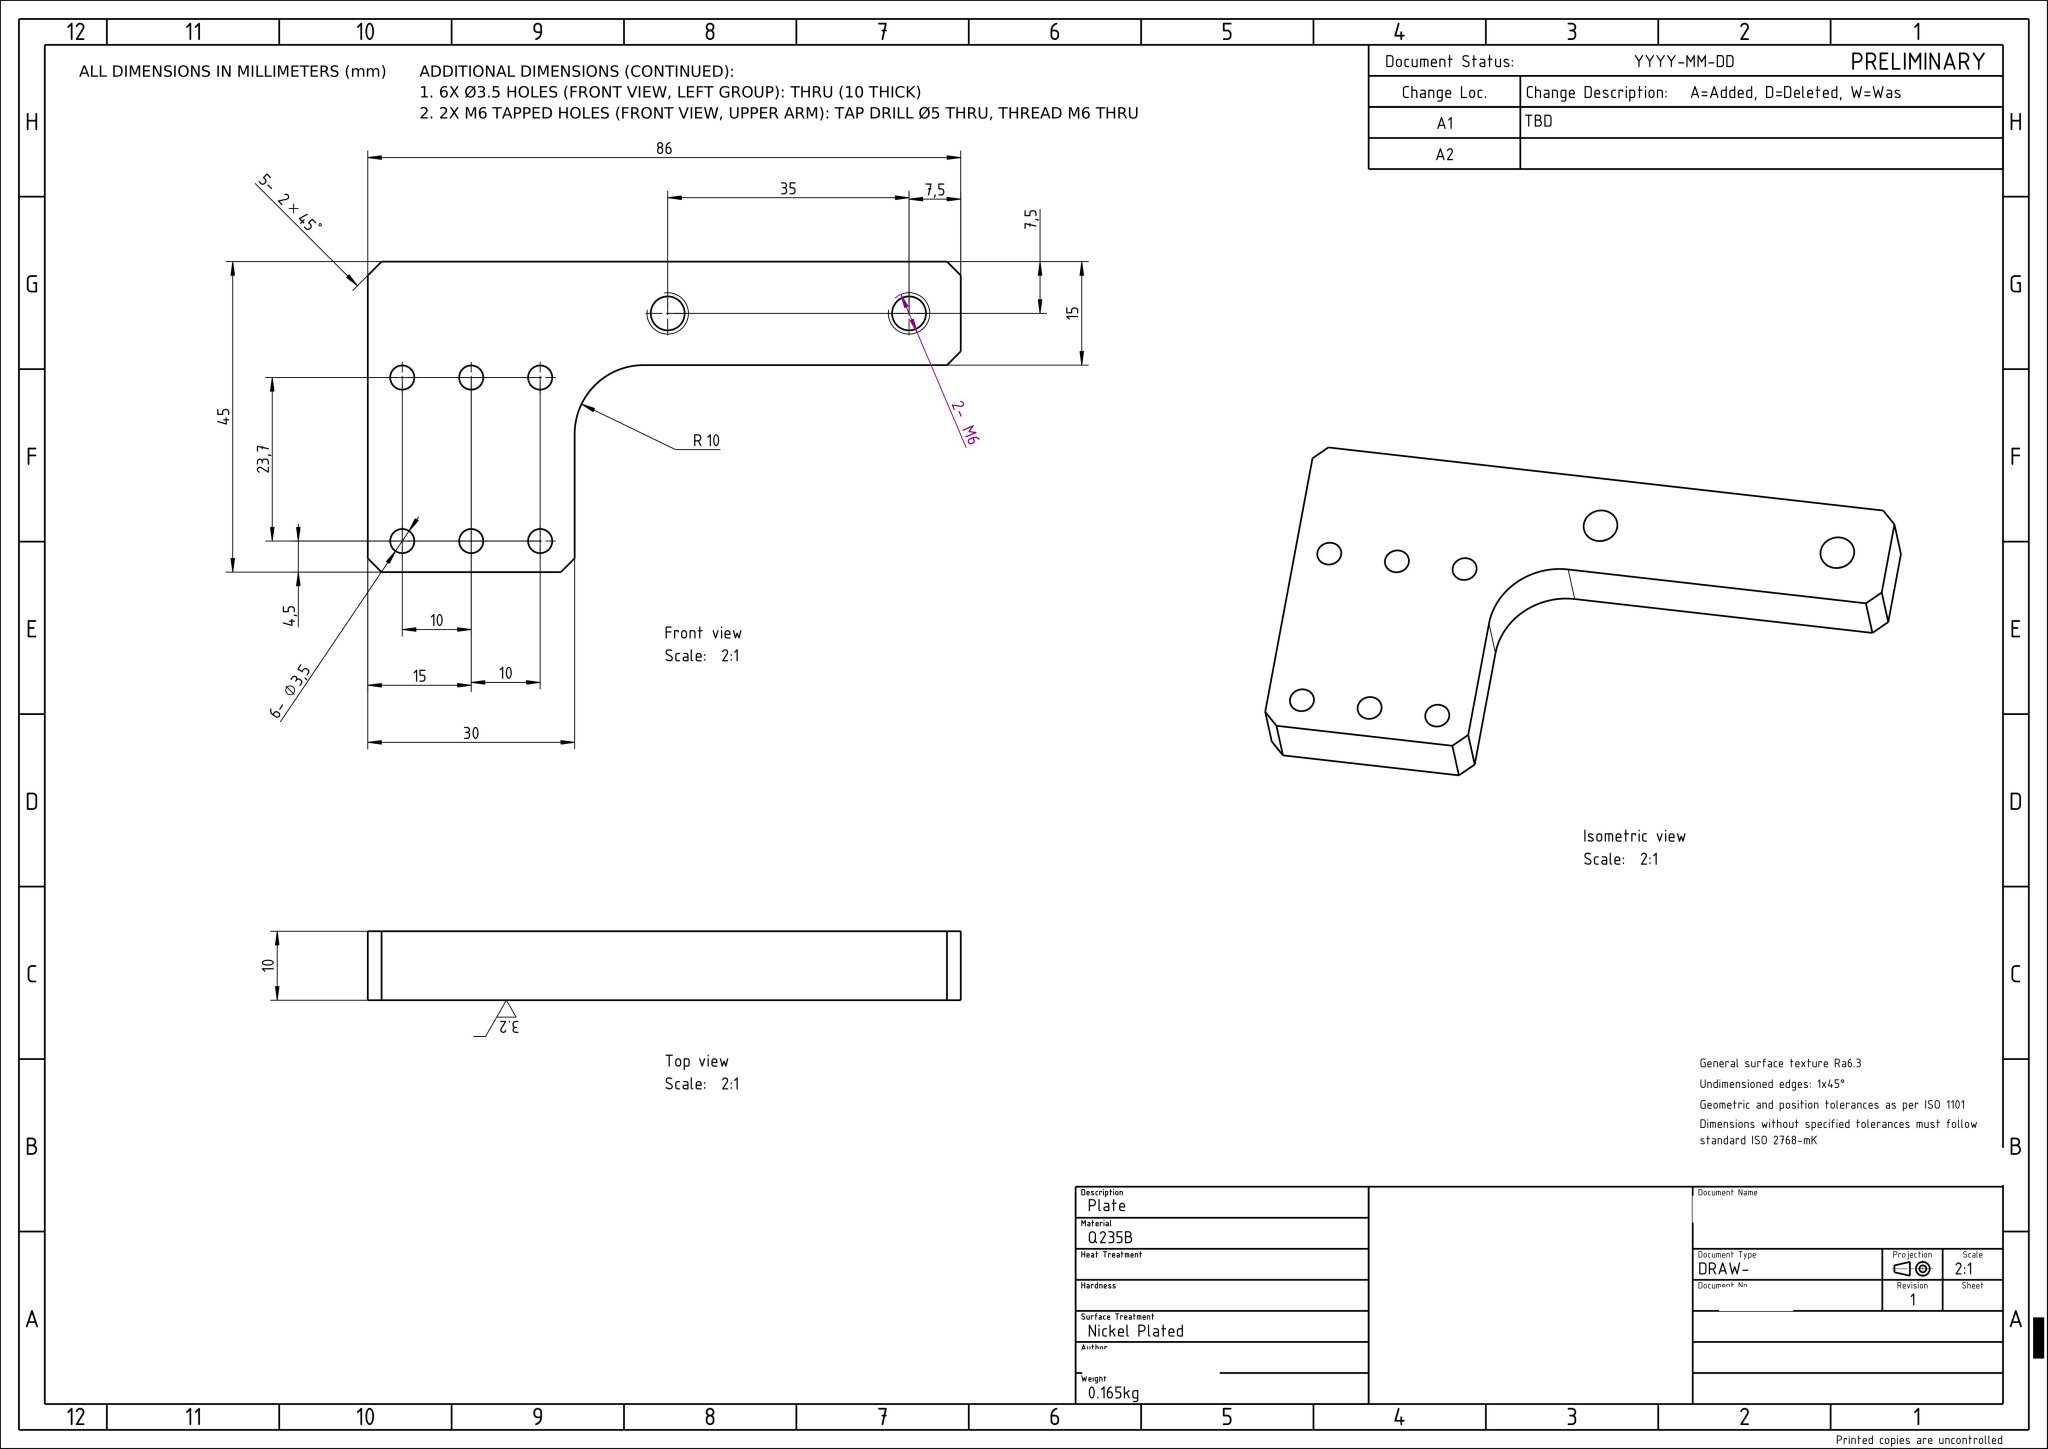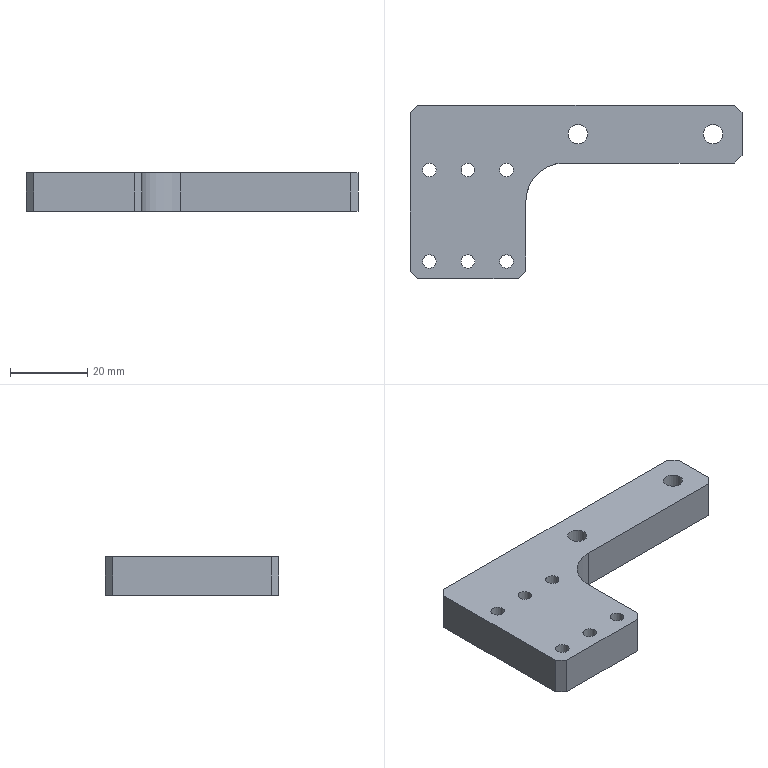Part | NX | mm | 1 solid | 22 faces | box 86 x 45 x 10 mm | volume 21045 mm3 | plane 13 | cylinder 9 | commonest cylinder face diameters 3.5 x6 5 x2 20 x1
STEP:
#1=CARTESIAN_POINT('',(0.,0.,0.));
#2=DIRECTION('',(0.,0.,1.));
#3=DIRECTION('',(1.,0.,0.));
#4=AXIS2_PLACEMENT_3D('',#1,#2,#3);
#5=(LENGTH_UNIT()NAMED_UNIT(*)SI_UNIT(.MILLI.,.METRE.));
#6=UNCERTAINTY_MEASURE_WITH_UNIT(LENGTH_MEASURE(0.00002),#5,'','');
#7=(NAMED_UNIT(*)PLANE_ANGLE_UNIT()SI_UNIT($,.RADIAN.));
#8=PLANE_ANGLE_MEASURE_WITH_UNIT(PLANE_ANGLE_MEASURE(0.01745),#7);
#9=DIMENSIONAL_EXPONENTS(0.,0.,0.,0.,0.,0.,0.);
#10=(CONVERSION_BASED_UNIT('',#8)NAMED_UNIT(#9)PLANE_ANGLE_UNIT());
#11=(NAMED_UNIT(*)SI_UNIT($,.STERADIAN.)SOLID_ANGLE_UNIT());
#12=(GEOMETRIC_REPRESENTATION_CONTEXT(3)GLOBAL_UNCERTAINTY_ASSIGNED_CONTEXT((#6))GLOBAL_UNIT_ASSIGNED_CONTEXT((#5,#10,#11))REPRESENTATION_CONTEXT('',''));
#13=SHAPE_REPRESENTATION('',(#4),#12);
#14=CARTESIAN_POINT('',(-15.,20.5,10.));
#15=VERTEX_POINT('',#14);
#16=CARTESIAN_POINT('',(-15.,-20.5,10.));
#17=VERTEX_POINT('',#16);
#18=CARTESIAN_POINT('',(-15.,22.5,10.));
#19=DIRECTION('',(-0.,-1.,0.));
#20=VECTOR('',#19,1.);
#21=LINE('',#18,#20);
#22=EDGE_CURVE('',#15,#17,#21,.T.);
#23=ORIENTED_EDGE('',*,*,#22,.F.);
#24=CARTESIAN_POINT('',(-15.,20.5,0.));
#25=VERTEX_POINT('',#24);
#26=CARTESIAN_POINT('',(-15.,20.5,10.));
#27=DIRECTION('',(0.,0.,-1.));
#28=VECTOR('',#27,1.);
#29=LINE('',#26,#28);
#30=EDGE_CURVE('',#15,#25,#29,.T.);
#31=ORIENTED_EDGE('',*,*,#30,.T.);
#32=CARTESIAN_POINT('',(-15.,-20.5,0.));
#33=VERTEX_POINT('',#32);
#34=CARTESIAN_POINT('',(-15.,22.5,0.));
#35=DIRECTION('',(-0.,-1.,0.));
#36=VECTOR('',#35,1.);
#37=LINE('',#34,#36);
#38=EDGE_CURVE('',#25,#33,#37,.T.);
#39=ORIENTED_EDGE('',*,*,#38,.T.);
#40=CARTESIAN_POINT('',(-15.,-20.5,10.));
#41=DIRECTION('',(0.,0.,1.));
#42=VECTOR('',#41,1.);
#43=LINE('',#40,#42);
#44=EDGE_CURVE('',#33,#17,#43,.T.);
#45=ORIENTED_EDGE('',*,*,#44,.T.);
#46=EDGE_LOOP('',(#23,#31,#39,#45));
#47=FACE_OUTER_BOUND('',#46,.T.);
#48=CARTESIAN_POINT('',(-15.,22.5,10.));
#49=DIRECTION('',(1.,-0.,0.));
#50=DIRECTION('',(0.,1.,0.));
#51=AXIS2_PLACEMENT_3D('',#48,#49,#50);
#52=PLANE('',#51);
#53=ADVANCED_FACE('',(#47),#52,.F.);
#54=CARTESIAN_POINT('',(-13.,-22.5,0.));
#55=VERTEX_POINT('',#54);
#56=CARTESIAN_POINT('',(13.,-22.5,0.));
#57=VERTEX_POINT('',#56);
#58=CARTESIAN_POINT('',(-15.,-22.5,0.));
#59=DIRECTION('',(1.,-0.,0.));
#60=VECTOR('',#59,1.);
#61=LINE('',#58,#60);
#62=EDGE_CURVE('',#55,#57,#61,.T.);
#63=ORIENTED_EDGE('',*,*,#62,.T.);
#64=CARTESIAN_POINT('',(13.,-22.5,10.));
#65=VERTEX_POINT('',#64);
#66=CARTESIAN_POINT('',(13.,-22.5,10.));
#67=DIRECTION('',(0.,0.,1.));
#68=VECTOR('',#67,1.);
#69=LINE('',#66,#68);
#70=EDGE_CURVE('',#57,#65,#69,.T.);
#71=ORIENTED_EDGE('',*,*,#70,.T.);
#72=CARTESIAN_POINT('',(-13.,-22.5,10.));
#73=VERTEX_POINT('',#72);
#74=CARTESIAN_POINT('',(-15.,-22.5,10.));
#75=DIRECTION('',(1.,-0.,0.));
#76=VECTOR('',#75,1.);
#77=LINE('',#74,#76);
#78=EDGE_CURVE('',#73,#65,#77,.T.);
#79=ORIENTED_EDGE('',*,*,#78,.F.);
#80=CARTESIAN_POINT('',(-13.,-22.5,10.));
#81=DIRECTION('',(0.,0.,-1.));
#82=VECTOR('',#81,1.);
#83=LINE('',#80,#82);
#84=EDGE_CURVE('',#73,#55,#83,.T.);
#85=ORIENTED_EDGE('',*,*,#84,.T.);
#86=EDGE_LOOP('',(#63,#71,#79,#85));
#87=FACE_OUTER_BOUND('',#86,.T.);
#88=CARTESIAN_POINT('',(-15.,-22.5,10.));
#89=DIRECTION('',(0.,1.,0.));
#90=DIRECTION('',(-1.,0.,0.));
#91=AXIS2_PLACEMENT_3D('',#88,#89,#90);
#92=PLANE('',#91);
#93=ADVANCED_FACE('',(#87),#92,.F.);
#94=CARTESIAN_POINT('',(15.,-20.5,10.));
#95=VERTEX_POINT('',#94);
#96=CARTESIAN_POINT('',(15.,-2.5,10.));
#97=VERTEX_POINT('',#96);
#98=CARTESIAN_POINT('',(15.,-22.5,10.));
#99=DIRECTION('',(0.,1.,0.));
#100=VECTOR('',#99,1.);
#101=LINE('',#98,#100);
#102=EDGE_CURVE('',#95,#97,#101,.T.);
#103=ORIENTED_EDGE('',*,*,#102,.F.);
#104=CARTESIAN_POINT('',(15.,-20.5,0.));
#105=VERTEX_POINT('',#104);
#106=CARTESIAN_POINT('',(15.,-20.5,10.));
#107=DIRECTION('',(0.,0.,-1.));
#108=VECTOR('',#107,1.);
#109=LINE('',#106,#108);
#110=EDGE_CURVE('',#95,#105,#109,.T.);
#111=ORIENTED_EDGE('',*,*,#110,.T.);
#112=CARTESIAN_POINT('',(15.,-2.5,0.));
#113=VERTEX_POINT('',#112);
#114=CARTESIAN_POINT('',(15.,-22.5,0.));
#115=DIRECTION('',(0.,1.,0.));
#116=VECTOR('',#115,1.);
#117=LINE('',#114,#116);
#118=EDGE_CURVE('',#105,#113,#117,.T.);
#119=ORIENTED_EDGE('',*,*,#118,.T.);
#120=CARTESIAN_POINT('',(15.,-2.5,10.));
#121=DIRECTION('',(0.,0.,1.));
#122=VECTOR('',#121,1.);
#123=LINE('',#120,#122);
#124=EDGE_CURVE('',#113,#97,#123,.T.);
#125=ORIENTED_EDGE('',*,*,#124,.T.);
#126=EDGE_LOOP('',(#103,#111,#119,#125));
#127=FACE_OUTER_BOUND('',#126,.T.);
#128=CARTESIAN_POINT('',(15.,-22.5,10.));
#129=DIRECTION('',(-1.,0.,0.));
#130=DIRECTION('',(0.,0.,1.));
#131=AXIS2_PLACEMENT_3D('',#128,#129,#130);
#132=PLANE('',#131);
#133=ADVANCED_FACE('',(#127),#132,.F.);
#134=CARTESIAN_POINT('',(25.,7.5,0.));
#135=VERTEX_POINT('',#134);
#136=CARTESIAN_POINT('',(69.,7.5,0.));
#137=VERTEX_POINT('',#136);
#138=CARTESIAN_POINT('',(15.,7.5,0.));
#139=DIRECTION('',(1.,-0.,0.));
#140=VECTOR('',#139,1.);
#141=LINE('',#138,#140);
#142=EDGE_CURVE('',#135,#137,#141,.T.);
#143=ORIENTED_EDGE('',*,*,#142,.T.);
#144=CARTESIAN_POINT('',(69.,7.5,10.));
#145=VERTEX_POINT('',#144);
#146=CARTESIAN_POINT('',(69.,7.5,10.));
#147=DIRECTION('',(0.,0.,1.));
#148=VECTOR('',#147,1.);
#149=LINE('',#146,#148);
#150=EDGE_CURVE('',#137,#145,#149,.T.);
#151=ORIENTED_EDGE('',*,*,#150,.T.);
#152=CARTESIAN_POINT('',(25.,7.5,10.));
#153=VERTEX_POINT('',#152);
#154=CARTESIAN_POINT('',(15.,7.5,10.));
#155=DIRECTION('',(1.,-0.,0.));
#156=VECTOR('',#155,1.);
#157=LINE('',#154,#156);
#158=EDGE_CURVE('',#153,#145,#157,.T.);
#159=ORIENTED_EDGE('',*,*,#158,.F.);
#160=CARTESIAN_POINT('',(25.,7.5,0.));
#161=DIRECTION('',(0.,0.,-1.));
#162=VECTOR('',#161,1.);
#163=LINE('',#160,#162);
#164=EDGE_CURVE('',#153,#135,#163,.T.);
#165=ORIENTED_EDGE('',*,*,#164,.T.);
#166=EDGE_LOOP('',(#143,#151,#159,#165));
#167=FACE_OUTER_BOUND('',#166,.T.);
#168=CARTESIAN_POINT('',(15.,7.5,10.));
#169=DIRECTION('',(0.,1.,0.));
#170=DIRECTION('',(-1.,0.,0.));
#171=AXIS2_PLACEMENT_3D('',#168,#169,#170);
#172=PLANE('',#171);
#173=ADVANCED_FACE('',(#167),#172,.F.);
#174=CARTESIAN_POINT('',(71.,9.5,0.));
#175=VERTEX_POINT('',#174);
#176=CARTESIAN_POINT('',(71.,20.5,0.));
#177=VERTEX_POINT('',#176);
#178=CARTESIAN_POINT('',(71.,7.5,0.));
#179=DIRECTION('',(0.,1.,0.));
#180=VECTOR('',#179,1.);
#181=LINE('',#178,#180);
#182=EDGE_CURVE('',#175,#177,#181,.T.);
#183=ORIENTED_EDGE('',*,*,#182,.T.);
#184=CARTESIAN_POINT('',(71.,20.5,10.));
#185=VERTEX_POINT('',#184);
#186=CARTESIAN_POINT('',(71.,20.5,10.));
#187=DIRECTION('',(0.,0.,1.));
#188=VECTOR('',#187,1.);
#189=LINE('',#186,#188);
#190=EDGE_CURVE('',#177,#185,#189,.T.);
#191=ORIENTED_EDGE('',*,*,#190,.T.);
#192=CARTESIAN_POINT('',(71.,9.5,10.));
#193=VERTEX_POINT('',#192);
#194=CARTESIAN_POINT('',(71.,7.5,10.));
#195=DIRECTION('',(0.,1.,0.));
#196=VECTOR('',#195,1.);
#197=LINE('',#194,#196);
#198=EDGE_CURVE('',#193,#185,#197,.T.);
#199=ORIENTED_EDGE('',*,*,#198,.F.);
#200=CARTESIAN_POINT('',(71.,9.5,10.));
#201=DIRECTION('',(0.,0.,-1.));
#202=VECTOR('',#201,1.);
#203=LINE('',#200,#202);
#204=EDGE_CURVE('',#193,#175,#203,.T.);
#205=ORIENTED_EDGE('',*,*,#204,.T.);
#206=EDGE_LOOP('',(#183,#191,#199,#205));
#207=FACE_OUTER_BOUND('',#206,.T.);
#208=CARTESIAN_POINT('',(71.,7.5,10.));
#209=DIRECTION('',(-1.,0.,0.));
#210=DIRECTION('',(0.,0.,1.));
#211=AXIS2_PLACEMENT_3D('',#208,#209,#210);
#212=PLANE('',#211);
#213=ADVANCED_FACE('',(#207),#212,.F.);
#214=CARTESIAN_POINT('',(69.,22.5,10.));
#215=VERTEX_POINT('',#214);
#216=CARTESIAN_POINT('',(-13.,22.5,10.));
#217=VERTEX_POINT('',#216);
#218=CARTESIAN_POINT('',(71.,22.5,10.));
#219=DIRECTION('',(-1.,0.,0.));
#220=VECTOR('',#219,1.);
#221=LINE('',#218,#220);
#222=EDGE_CURVE('',#215,#217,#221,.T.);
#223=ORIENTED_EDGE('',*,*,#222,.F.);
#224=CARTESIAN_POINT('',(69.,22.5,0.));
#225=VERTEX_POINT('',#224);
#226=CARTESIAN_POINT('',(69.,22.5,10.));
#227=DIRECTION('',(0.,0.,-1.));
#228=VECTOR('',#227,1.);
#229=LINE('',#226,#228);
#230=EDGE_CURVE('',#215,#225,#229,.T.);
#231=ORIENTED_EDGE('',*,*,#230,.T.);
#232=CARTESIAN_POINT('',(-13.,22.5,0.));
#233=VERTEX_POINT('',#232);
#234=CARTESIAN_POINT('',(71.,22.5,0.));
#235=DIRECTION('',(-1.,0.,0.));
#236=VECTOR('',#235,1.);
#237=LINE('',#234,#236);
#238=EDGE_CURVE('',#225,#233,#237,.T.);
#239=ORIENTED_EDGE('',*,*,#238,.T.);
#240=CARTESIAN_POINT('',(-13.,22.5,10.));
#241=DIRECTION('',(0.,0.,1.));
#242=VECTOR('',#241,1.);
#243=LINE('',#240,#242);
#244=EDGE_CURVE('',#233,#217,#243,.T.);
#245=ORIENTED_EDGE('',*,*,#244,.T.);
#246=EDGE_LOOP('',(#223,#231,#239,#245));
#247=FACE_OUTER_BOUND('',#246,.T.);
#248=CARTESIAN_POINT('',(71.,22.5,10.));
#249=DIRECTION('',(0.,-1.,0.));
#250=DIRECTION('',(0.,0.,-1.));
#251=AXIS2_PLACEMENT_3D('',#248,#249,#250);
#252=PLANE('',#251);
#253=ADVANCED_FACE('',(#247),#252,.F.);
#254=CARTESIAN_POINT('',(8.25,5.7,10.));
#255=VERTEX_POINT('',#254);
#256=CARTESIAN_POINT('',(10.,5.7,10.));
#257=DIRECTION('',(0.,0.,-1.));
#258=DIRECTION('',(-1.,0.,0.));
#259=AXIS2_PLACEMENT_3D('',#256,#257,#258);
#260=CIRCLE('',#259,1.75);
#261=EDGE_CURVE('',#255,#255,#260,.T.);
#262=ORIENTED_EDGE('',*,*,#261,.T.);
#263=EDGE_LOOP('',(#262));
#264=FACE_BOUND('',#263,.T.);
#265=CARTESIAN_POINT('',(8.25,-18.,10.));
#266=VERTEX_POINT('',#265);
#267=CARTESIAN_POINT('',(10.,-18.,10.));
#268=DIRECTION('',(0.,0.,-1.));
#269=DIRECTION('',(-1.,0.,0.));
#270=AXIS2_PLACEMENT_3D('',#267,#268,#269);
#271=CIRCLE('',#270,1.75);
#272=EDGE_CURVE('',#266,#266,#271,.T.);
#273=ORIENTED_EDGE('',*,*,#272,.T.);
#274=EDGE_LOOP('',(#273));
#275=FACE_BOUND('',#274,.T.);
#276=CARTESIAN_POINT('',(-1.75,5.7,10.));
#277=VERTEX_POINT('',#276);
#278=CARTESIAN_POINT('',(0.,5.7,10.));
#279=DIRECTION('',(0.,0.,-1.));
#280=DIRECTION('',(-1.,0.,0.));
#281=AXIS2_PLACEMENT_3D('',#278,#279,#280);
#282=CIRCLE('',#281,1.75);
#283=EDGE_CURVE('',#277,#277,#282,.T.);
#284=ORIENTED_EDGE('',*,*,#283,.T.);
#285=EDGE_LOOP('',(#284));
#286=FACE_BOUND('',#285,.T.);
#287=CARTESIAN_POINT('',(-1.75,-18.,10.));
#288=VERTEX_POINT('',#287);
#289=CARTESIAN_POINT('',(0.,-18.,10.));
#290=DIRECTION('',(0.,0.,-1.));
#291=DIRECTION('',(-1.,0.,0.));
#292=AXIS2_PLACEMENT_3D('',#289,#290,#291);
#293=CIRCLE('',#292,1.75);
#294=EDGE_CURVE('',#288,#288,#293,.T.);
#295=ORIENTED_EDGE('',*,*,#294,.T.);
#296=EDGE_LOOP('',(#295));
#297=FACE_BOUND('',#296,.T.);
#298=CARTESIAN_POINT('',(-11.75,5.7,10.));
#299=VERTEX_POINT('',#298);
#300=CARTESIAN_POINT('',(-10.,5.7,10.));
#301=DIRECTION('',(0.,0.,-1.));
#302=DIRECTION('',(-1.,0.,0.));
#303=AXIS2_PLACEMENT_3D('',#300,#301,#302);
#304=CIRCLE('',#303,1.75);
#305=EDGE_CURVE('',#299,#299,#304,.T.);
#306=ORIENTED_EDGE('',*,*,#305,.T.);
#307=EDGE_LOOP('',(#306));
#308=FACE_BOUND('',#307,.T.);
#309=CARTESIAN_POINT('',(-11.75,-18.,10.));
#310=VERTEX_POINT('',#309);
#311=CARTESIAN_POINT('',(-10.,-18.,10.));
#312=DIRECTION('',(0.,0.,-1.));
#313=DIRECTION('',(-1.,0.,0.));
#314=AXIS2_PLACEMENT_3D('',#311,#312,#313);
#315=CIRCLE('',#314,1.75);
#316=EDGE_CURVE('',#310,#310,#315,.T.);
#317=ORIENTED_EDGE('',*,*,#316,.T.);
#318=EDGE_LOOP('',(#317));
#319=FACE_BOUND('',#318,.T.);
#320=CARTESIAN_POINT('',(61.,15.,10.));
#321=VERTEX_POINT('',#320);
#322=CARTESIAN_POINT('',(63.5,15.,10.));
#323=DIRECTION('',(0.,0.,-1.));
#324=DIRECTION('',(-1.,0.,0.));
#325=AXIS2_PLACEMENT_3D('',#322,#323,#324);
#326=CIRCLE('',#325,2.5);
#327=EDGE_CURVE('',#321,#321,#326,.T.);
#328=ORIENTED_EDGE('',*,*,#327,.T.);
#329=EDGE_LOOP('',(#328));
#330=FACE_BOUND('',#329,.T.);
#331=CARTESIAN_POINT('',(26.,15.,10.));
#332=VERTEX_POINT('',#331);
#333=CARTESIAN_POINT('',(28.5,15.,10.));
#334=DIRECTION('',(0.,0.,-1.));
#335=DIRECTION('',(-1.,0.,0.));
#336=AXIS2_PLACEMENT_3D('',#333,#334,#335);
#337=CIRCLE('',#336,2.5);
#338=EDGE_CURVE('',#332,#332,#337,.T.);
#339=ORIENTED_EDGE('',*,*,#338,.T.);
#340=EDGE_LOOP('',(#339));
#341=FACE_BOUND('',#340,.T.);
#342=ORIENTED_EDGE('',*,*,#198,.T.);
#343=CARTESIAN_POINT('',(45.75,45.75,10.));
#344=DIRECTION('',(-0.7071,0.7071,0.));
#345=VECTOR('',#344,1.);
#346=LINE('',#343,#345);
#347=EDGE_CURVE('',#185,#215,#346,.T.);
#348=ORIENTED_EDGE('',*,*,#347,.T.);
#349=ORIENTED_EDGE('',*,*,#222,.T.);
#350=CARTESIAN_POINT('',(-17.75,17.75,10.));
#351=DIRECTION('',(-0.7071,-0.7071,0.));
#352=VECTOR('',#351,1.);
#353=LINE('',#350,#352);
#354=EDGE_CURVE('',#217,#15,#353,.T.);
#355=ORIENTED_EDGE('',*,*,#354,.T.);
#356=ORIENTED_EDGE('',*,*,#22,.T.);
#357=CARTESIAN_POINT('',(-17.75,-17.75,10.));
#358=DIRECTION('',(0.7071,-0.7071,0.));
#359=VECTOR('',#358,1.);
#360=LINE('',#357,#359);
#361=EDGE_CURVE('',#17,#73,#360,.T.);
#362=ORIENTED_EDGE('',*,*,#361,.T.);
#363=ORIENTED_EDGE('',*,*,#78,.T.);
#364=CARTESIAN_POINT('',(17.75,-17.75,10.));
#365=DIRECTION('',(0.7071,0.7071,0.));
#366=VECTOR('',#365,1.);
#367=LINE('',#364,#366);
#368=EDGE_CURVE('',#65,#95,#367,.T.);
#369=ORIENTED_EDGE('',*,*,#368,.T.);
#370=ORIENTED_EDGE('',*,*,#102,.T.);
#371=CARTESIAN_POINT('',(25.,-2.5,10.));
#372=DIRECTION('',(0.,0.,-1.));
#373=DIRECTION('',(1.,0.,0.));
#374=AXIS2_PLACEMENT_3D('',#371,#372,#373);
#375=CIRCLE('',#374,10.);
#376=EDGE_CURVE('',#97,#153,#375,.T.);
#377=ORIENTED_EDGE('',*,*,#376,.T.);
#378=ORIENTED_EDGE('',*,*,#158,.T.);
#379=CARTESIAN_POINT('',(30.75,-30.75,10.));
#380=DIRECTION('',(0.7071,0.7071,0.));
#381=VECTOR('',#380,1.);
#382=LINE('',#379,#381);
#383=EDGE_CURVE('',#145,#193,#382,.T.);
#384=ORIENTED_EDGE('',*,*,#383,.T.);
#385=EDGE_LOOP('',(#342,#348,#349,#355,#356,#362,#363,#369,#370,#377,#378,#384));
#386=FACE_BOUND('',#385,.T.);
#387=CARTESIAN_POINT('',(0.,0.,10.));
#388=DIRECTION('',(0.,0.,1.));
#389=DIRECTION('',(1.,0.,0.));
#390=AXIS2_PLACEMENT_3D('',#387,#388,#389);
#391=PLANE('',#390);
#392=ADVANCED_FACE('',(#264,#275,#286,#297,#308,#319,#330,#341,#386),#391,.T.);
#393=CARTESIAN_POINT('',(11.75,5.7,0.));
#394=VERTEX_POINT('',#393);
#395=CARTESIAN_POINT('',(10.,5.7,0.));
#396=DIRECTION('',(0.,0.,1.));
#397=DIRECTION('',(1.,0.,0.));
#398=AXIS2_PLACEMENT_3D('',#395,#396,#397);
#399=CIRCLE('',#398,1.75);
#400=EDGE_CURVE('',#394,#394,#399,.T.);
#401=ORIENTED_EDGE('',*,*,#400,.T.);
#402=EDGE_LOOP('',(#401));
#403=FACE_BOUND('',#402,.T.);
#404=CARTESIAN_POINT('',(11.75,-18.,0.));
#405=VERTEX_POINT('',#404);
#406=CARTESIAN_POINT('',(10.,-18.,0.));
#407=DIRECTION('',(0.,0.,1.));
#408=DIRECTION('',(1.,0.,0.));
#409=AXIS2_PLACEMENT_3D('',#406,#407,#408);
#410=CIRCLE('',#409,1.75);
#411=EDGE_CURVE('',#405,#405,#410,.T.);
#412=ORIENTED_EDGE('',*,*,#411,.T.);
#413=EDGE_LOOP('',(#412));
#414=FACE_BOUND('',#413,.T.);
#415=CARTESIAN_POINT('',(1.75,5.7,0.));
#416=VERTEX_POINT('',#415);
#417=CARTESIAN_POINT('',(0.,5.7,0.));
#418=DIRECTION('',(0.,0.,1.));
#419=DIRECTION('',(1.,0.,0.));
#420=AXIS2_PLACEMENT_3D('',#417,#418,#419);
#421=CIRCLE('',#420,1.75);
#422=EDGE_CURVE('',#416,#416,#421,.T.);
#423=ORIENTED_EDGE('',*,*,#422,.T.);
#424=EDGE_LOOP('',(#423));
#425=FACE_BOUND('',#424,.T.);
#426=CARTESIAN_POINT('',(1.75,-18.,0.));
#427=VERTEX_POINT('',#426);
#428=CARTESIAN_POINT('',(0.,-18.,0.));
#429=DIRECTION('',(0.,0.,1.));
#430=DIRECTION('',(1.,0.,0.));
#431=AXIS2_PLACEMENT_3D('',#428,#429,#430);
#432=CIRCLE('',#431,1.75);
#433=EDGE_CURVE('',#427,#427,#432,.T.);
#434=ORIENTED_EDGE('',*,*,#433,.T.);
#435=EDGE_LOOP('',(#434));
#436=FACE_BOUND('',#435,.T.);
#437=CARTESIAN_POINT('',(-8.25,5.7,0.));
#438=VERTEX_POINT('',#437);
#439=CARTESIAN_POINT('',(-10.,5.7,0.));
#440=DIRECTION('',(0.,0.,1.));
#441=DIRECTION('',(1.,0.,0.));
#442=AXIS2_PLACEMENT_3D('',#439,#440,#441);
#443=CIRCLE('',#442,1.75);
#444=EDGE_CURVE('',#438,#438,#443,.T.);
#445=ORIENTED_EDGE('',*,*,#444,.T.);
#446=EDGE_LOOP('',(#445));
#447=FACE_BOUND('',#446,.T.);
#448=CARTESIAN_POINT('',(-8.25,-18.,0.));
#449=VERTEX_POINT('',#448);
#450=CARTESIAN_POINT('',(-10.,-18.,0.));
#451=DIRECTION('',(0.,0.,1.));
#452=DIRECTION('',(1.,0.,0.));
#453=AXIS2_PLACEMENT_3D('',#450,#451,#452);
#454=CIRCLE('',#453,1.75);
#455=EDGE_CURVE('',#449,#449,#454,.T.);
#456=ORIENTED_EDGE('',*,*,#455,.T.);
#457=EDGE_LOOP('',(#456));
#458=FACE_BOUND('',#457,.T.);
#459=CARTESIAN_POINT('',(66.,15.,0.));
#460=VERTEX_POINT('',#459);
#461=CARTESIAN_POINT('',(63.5,15.,0.));
#462=DIRECTION('',(0.,0.,1.));
#463=DIRECTION('',(1.,0.,0.));
#464=AXIS2_PLACEMENT_3D('',#461,#462,#463);
#465=CIRCLE('',#464,2.5);
#466=EDGE_CURVE('',#460,#460,#465,.T.);
#467=ORIENTED_EDGE('',*,*,#466,.T.);
#468=EDGE_LOOP('',(#467));
#469=FACE_BOUND('',#468,.T.);
#470=CARTESIAN_POINT('',(31.,15.,0.));
#471=VERTEX_POINT('',#470);
#472=CARTESIAN_POINT('',(28.5,15.,0.));
#473=DIRECTION('',(0.,0.,1.));
#474=DIRECTION('',(1.,0.,0.));
#475=AXIS2_PLACEMENT_3D('',#472,#473,#474);
#476=CIRCLE('',#475,2.5);
#477=EDGE_CURVE('',#471,#471,#476,.T.);
#478=ORIENTED_EDGE('',*,*,#477,.T.);
#479=EDGE_LOOP('',(#478));
#480=FACE_BOUND('',#479,.T.);
#481=ORIENTED_EDGE('',*,*,#238,.F.);
#482=CARTESIAN_POINT('',(69.,22.5,0.));
#483=DIRECTION('',(0.7071,-0.7071,0.));
#484=VECTOR('',#483,1.);
#485=LINE('',#482,#484);
#486=EDGE_CURVE('',#225,#177,#485,.T.);
#487=ORIENTED_EDGE('',*,*,#486,.T.);
#488=ORIENTED_EDGE('',*,*,#182,.F.);
#489=CARTESIAN_POINT('',(71.,9.5,0.));
#490=DIRECTION('',(-0.7071,-0.7071,0.));
#491=VECTOR('',#490,1.);
#492=LINE('',#489,#491);
#493=EDGE_CURVE('',#175,#137,#492,.T.);
#494=ORIENTED_EDGE('',*,*,#493,.T.);
#495=ORIENTED_EDGE('',*,*,#142,.F.);
#496=CARTESIAN_POINT('',(25.,-2.5,0.));
#497=DIRECTION('',(0.,0.,1.));
#498=DIRECTION('',(1.,0.,0.));
#499=AXIS2_PLACEMENT_3D('',#496,#497,#498);
#500=CIRCLE('',#499,10.);
#501=EDGE_CURVE('',#135,#113,#500,.T.);
#502=ORIENTED_EDGE('',*,*,#501,.T.);
#503=ORIENTED_EDGE('',*,*,#118,.F.);
#504=CARTESIAN_POINT('',(15.,-20.5,0.));
#505=DIRECTION('',(-0.7071,-0.7071,0.));
#506=VECTOR('',#505,1.);
#507=LINE('',#504,#506);
#508=EDGE_CURVE('',#105,#57,#507,.T.);
#509=ORIENTED_EDGE('',*,*,#508,.T.);
#510=ORIENTED_EDGE('',*,*,#62,.F.);
#511=CARTESIAN_POINT('',(-13.,-22.5,0.));
#512=DIRECTION('',(-0.7071,0.7071,0.));
#513=VECTOR('',#512,1.);
#514=LINE('',#511,#513);
#515=EDGE_CURVE('',#55,#33,#514,.T.);
#516=ORIENTED_EDGE('',*,*,#515,.T.);
#517=ORIENTED_EDGE('',*,*,#38,.F.);
#518=CARTESIAN_POINT('',(-15.,20.5,0.));
#519=DIRECTION('',(0.7071,0.7071,0.));
#520=VECTOR('',#519,1.);
#521=LINE('',#518,#520);
#522=EDGE_CURVE('',#25,#233,#521,.T.);
#523=ORIENTED_EDGE('',*,*,#522,.T.);
#524=EDGE_LOOP('',(#481,#487,#488,#494,#495,#502,#503,#509,#510,#516,#517,#523));
#525=FACE_BOUND('',#524,.T.);
#526=CARTESIAN_POINT('',(0.,0.,0.));
#527=DIRECTION('',(0.,0.,1.));
#528=DIRECTION('',(1.,0.,0.));
#529=AXIS2_PLACEMENT_3D('',#526,#527,#528);
#530=PLANE('',#529);
#531=ADVANCED_FACE('',(#403,#414,#425,#436,#447,#458,#469,#480,#525),#530,.F.);
#532=ORIENTED_EDGE('',*,*,#376,.F.);
#533=ORIENTED_EDGE('',*,*,#124,.F.);
#534=ORIENTED_EDGE('',*,*,#501,.F.);
#535=ORIENTED_EDGE('',*,*,#164,.F.);
#536=EDGE_LOOP('',(#532,#533,#534,#535));
#537=FACE_OUTER_BOUND('',#536,.T.);
#538=CARTESIAN_POINT('',(25.,-2.5,10.));
#539=DIRECTION('',(0.,0.,1.));
#540=DIRECTION('',(1.,0.,0.));
#541=AXIS2_PLACEMENT_3D('',#538,#539,#540);
#542=CYLINDRICAL_SURFACE('',#541,10.);
#543=ADVANCED_FACE('',(#537),#542,.F.);
#544=ORIENTED_EDGE('',*,*,#347,.F.);
#545=ORIENTED_EDGE('',*,*,#190,.F.);
#546=ORIENTED_EDGE('',*,*,#486,.F.);
#547=ORIENTED_EDGE('',*,*,#230,.F.);
#548=EDGE_LOOP('',(#544,#545,#546,#547));
#549=FACE_OUTER_BOUND('',#548,.T.);
#550=CARTESIAN_POINT('',(69.,22.5,10.));
#551=DIRECTION('',(-0.7071,-0.7071,0.));
#552=DIRECTION('',(0.,0.,-1.));
#553=AXIS2_PLACEMENT_3D('',#550,#551,#552);
#554=PLANE('',#553);
#555=ADVANCED_FACE('',(#549),#554,.F.);
#556=ORIENTED_EDGE('',*,*,#383,.F.);
#557=ORIENTED_EDGE('',*,*,#150,.F.);
#558=ORIENTED_EDGE('',*,*,#493,.F.);
#559=ORIENTED_EDGE('',*,*,#204,.F.);
#560=EDGE_LOOP('',(#556,#557,#558,#559));
#561=FACE_OUTER_BOUND('',#560,.T.);
#562=CARTESIAN_POINT('',(71.,9.5,10.));
#563=DIRECTION('',(-0.7071,0.7071,0.));
#564=DIRECTION('',(0.,0.,-1.));
#565=AXIS2_PLACEMENT_3D('',#562,#563,#564);
#566=PLANE('',#565);
#567=ADVANCED_FACE('',(#561),#566,.F.);
#568=ORIENTED_EDGE('',*,*,#354,.F.);
#569=ORIENTED_EDGE('',*,*,#244,.F.);
#570=ORIENTED_EDGE('',*,*,#522,.F.);
#571=ORIENTED_EDGE('',*,*,#30,.F.);
#572=EDGE_LOOP('',(#568,#569,#570,#571));
#573=FACE_OUTER_BOUND('',#572,.T.);
#574=CARTESIAN_POINT('',(-15.,20.5,10.));
#575=DIRECTION('',(0.7071,-0.7071,0.));
#576=DIRECTION('',(0.,0.,-1.));
#577=AXIS2_PLACEMENT_3D('',#574,#575,#576);
#578=PLANE('',#577);
#579=ADVANCED_FACE('',(#573),#578,.F.);
#580=ORIENTED_EDGE('',*,*,#368,.F.);
#581=ORIENTED_EDGE('',*,*,#70,.F.);
#582=ORIENTED_EDGE('',*,*,#508,.F.);
#583=ORIENTED_EDGE('',*,*,#110,.F.);
#584=EDGE_LOOP('',(#580,#581,#582,#583));
#585=FACE_OUTER_BOUND('',#584,.T.);
#586=CARTESIAN_POINT('',(15.,-20.5,10.));
#587=DIRECTION('',(-0.7071,0.7071,0.));
#588=DIRECTION('',(0.,0.,-1.));
#589=AXIS2_PLACEMENT_3D('',#586,#587,#588);
#590=PLANE('',#589);
#591=ADVANCED_FACE('',(#585),#590,.F.);
#592=ORIENTED_EDGE('',*,*,#361,.F.);
#593=ORIENTED_EDGE('',*,*,#44,.F.);
#594=ORIENTED_EDGE('',*,*,#515,.F.);
#595=ORIENTED_EDGE('',*,*,#84,.F.);
#596=EDGE_LOOP('',(#592,#593,#594,#595));
#597=FACE_OUTER_BOUND('',#596,.T.);
#598=CARTESIAN_POINT('',(-13.,-22.5,10.));
#599=DIRECTION('',(0.7071,0.7071,0.));
#600=DIRECTION('',(0.,0.,-1.));
#601=AXIS2_PLACEMENT_3D('',#598,#599,#600);
#602=PLANE('',#601);
#603=ADVANCED_FACE('',(#597),#602,.F.);
#604=ORIENTED_EDGE('',*,*,#338,.F.);
#605=EDGE_LOOP('',(#604));
#606=FACE_BOUND('',#605,.T.);
#607=ORIENTED_EDGE('',*,*,#477,.F.);
#608=EDGE_LOOP('',(#607));
#609=FACE_BOUND('',#608,.T.);
#610=CARTESIAN_POINT('',(28.5,15.,10.));
#611=DIRECTION('',(0.,0.,-1.));
#612=DIRECTION('',(-1.,0.,0.));
#613=AXIS2_PLACEMENT_3D('',#610,#611,#612);
#614=CYLINDRICAL_SURFACE('',#613,2.5);
#615=ADVANCED_FACE('',(#606,#609),#614,.F.);
#616=ORIENTED_EDGE('',*,*,#327,.F.);
#617=EDGE_LOOP('',(#616));
#618=FACE_BOUND('',#617,.T.);
#619=ORIENTED_EDGE('',*,*,#466,.F.);
#620=EDGE_LOOP('',(#619));
#621=FACE_BOUND('',#620,.T.);
#622=CARTESIAN_POINT('',(63.5,15.,10.));
#623=DIRECTION('',(0.,0.,-1.));
#624=DIRECTION('',(-1.,0.,0.));
#625=AXIS2_PLACEMENT_3D('',#622,#623,#624);
#626=CYLINDRICAL_SURFACE('',#625,2.5);
#627=ADVANCED_FACE('',(#618,#621),#626,.F.);
#628=ORIENTED_EDGE('',*,*,#316,.F.);
#629=EDGE_LOOP('',(#628));
#630=FACE_BOUND('',#629,.T.);
#631=ORIENTED_EDGE('',*,*,#455,.F.);
#632=EDGE_LOOP('',(#631));
#633=FACE_BOUND('',#632,.T.);
#634=CARTESIAN_POINT('',(-10.,-18.,10.));
#635=DIRECTION('',(0.,0.,-1.));
#636=DIRECTION('',(-1.,0.,0.));
#637=AXIS2_PLACEMENT_3D('',#634,#635,#636);
#638=CYLINDRICAL_SURFACE('',#637,1.75);
#639=ADVANCED_FACE('',(#630,#633),#638,.F.);
#640=ORIENTED_EDGE('',*,*,#305,.F.);
#641=EDGE_LOOP('',(#640));
#642=FACE_BOUND('',#641,.T.);
#643=ORIENTED_EDGE('',*,*,#444,.F.);
#644=EDGE_LOOP('',(#643));
#645=FACE_BOUND('',#644,.T.);
#646=CARTESIAN_POINT('',(-10.,5.7,10.));
#647=DIRECTION('',(0.,0.,-1.));
#648=DIRECTION('',(-1.,0.,0.));
#649=AXIS2_PLACEMENT_3D('',#646,#647,#648);
#650=CYLINDRICAL_SURFACE('',#649,1.75);
#651=ADVANCED_FACE('',(#642,#645),#650,.F.);
#652=ORIENTED_EDGE('',*,*,#294,.F.);
#653=EDGE_LOOP('',(#652));
#654=FACE_BOUND('',#653,.T.);
#655=ORIENTED_EDGE('',*,*,#433,.F.);
#656=EDGE_LOOP('',(#655));
#657=FACE_BOUND('',#656,.T.);
#658=CARTESIAN_POINT('',(0.,-18.,10.));
#659=DIRECTION('',(0.,0.,-1.));
#660=DIRECTION('',(-1.,0.,0.));
#661=AXIS2_PLACEMENT_3D('',#658,#659,#660);
#662=CYLINDRICAL_SURFACE('',#661,1.75);
#663=ADVANCED_FACE('',(#654,#657),#662,.F.);
#664=ORIENTED_EDGE('',*,*,#283,.F.);
#665=EDGE_LOOP('',(#664));
#666=FACE_BOUND('',#665,.T.);
#667=ORIENTED_EDGE('',*,*,#422,.F.);
#668=EDGE_LOOP('',(#667));
#669=FACE_BOUND('',#668,.T.);
#670=CARTESIAN_POINT('',(0.,5.7,10.));
#671=DIRECTION('',(0.,0.,-1.));
#672=DIRECTION('',(-1.,0.,0.));
#673=AXIS2_PLACEMENT_3D('',#670,#671,#672);
#674=CYLINDRICAL_SURFACE('',#673,1.75);
#675=ADVANCED_FACE('',(#666,#669),#674,.F.);
#676=ORIENTED_EDGE('',*,*,#272,.F.);
#677=EDGE_LOOP('',(#676));
#678=FACE_BOUND('',#677,.T.);
#679=ORIENTED_EDGE('',*,*,#411,.F.);
#680=EDGE_LOOP('',(#679));
#681=FACE_BOUND('',#680,.T.);
#682=CARTESIAN_POINT('',(10.,-18.,10.));
#683=DIRECTION('',(0.,0.,-1.));
#684=DIRECTION('',(-1.,0.,0.));
#685=AXIS2_PLACEMENT_3D('',#682,#683,#684);
#686=CYLINDRICAL_SURFACE('',#685,1.75);
#687=ADVANCED_FACE('',(#678,#681),#686,.F.);
#688=ORIENTED_EDGE('',*,*,#261,.F.);
#689=EDGE_LOOP('',(#688));
#690=FACE_BOUND('',#689,.T.);
#691=ORIENTED_EDGE('',*,*,#400,.F.);
#692=EDGE_LOOP('',(#691));
#693=FACE_BOUND('',#692,.T.);
#694=CARTESIAN_POINT('',(10.,5.7,10.));
#695=DIRECTION('',(0.,0.,-1.));
#696=DIRECTION('',(-1.,0.,0.));
#697=AXIS2_PLACEMENT_3D('',#694,#695,#696);
#698=CYLINDRICAL_SURFACE('',#697,1.75);
#699=ADVANCED_FACE('',(#690,#693),#698,.F.);
#700=CLOSED_SHELL('',(#53,#93,#133,#173,#213,#253,#392,#531,#543,#555,#567,#579,#591,#603,#615,#627,#639,#651,#663,#675,#687,#699));
#701=MANIFOLD_SOLID_BREP('',#700);
#702=ADVANCED_BREP_SHAPE_REPRESENTATION('',(#701),#12);
#703=SHAPE_REPRESENTATION_RELATIONSHIP('','',#13,#702);
#704=PRESENTATION_LAYER_ASSIGNMENT('','',(#701));
#705=COLOUR_RGB('',0.4,0.8,1.);
#706=FILL_AREA_STYLE_COLOUR('',#705);
#707=FILL_AREA_STYLE('',(#706));
#708=SURFACE_STYLE_FILL_AREA(#707);
#709=SURFACE_SIDE_STYLE('',(#708));
#710=SURFACE_STYLE_USAGE(.BOTH.,#709);
#711=PRESENTATION_STYLE_ASSIGNMENT((#710));
#712=STYLED_ITEM('',(#711),#701);
#713=MECHANICAL_DESIGN_GEOMETRIC_PRESENTATION_REPRESENTATION('',(#712),#12);